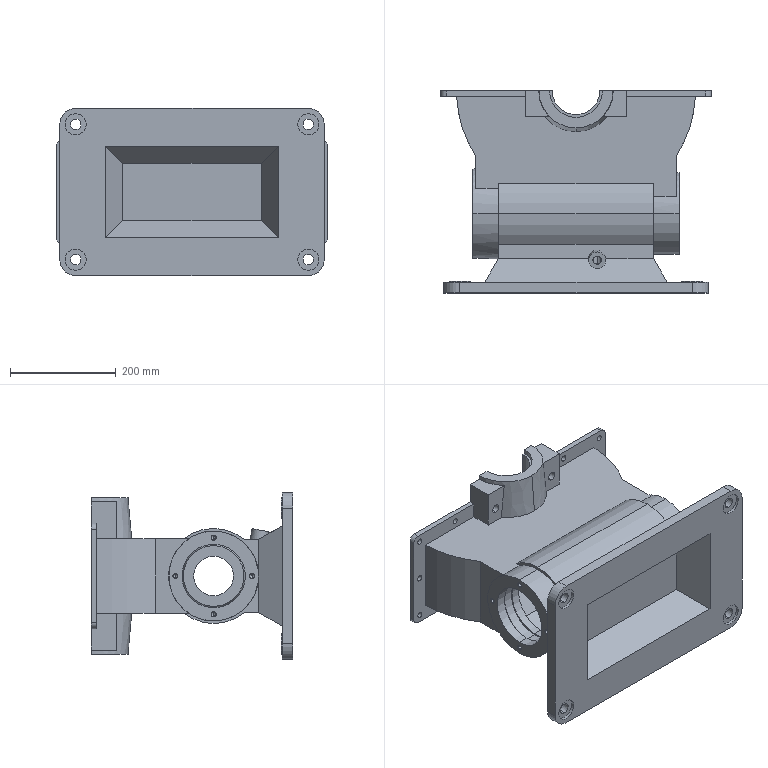Component | SolidWorks | 2Housing-1 | 1 solid | 226 faces | volume 9015578 mm3 | cylinder 110 | plane 74 | cone 42 | commonest cylinder face diameters 11 x20 40 x16 8.5 x16 16 x8 20 x8 120 x4 24 x4 60 x4